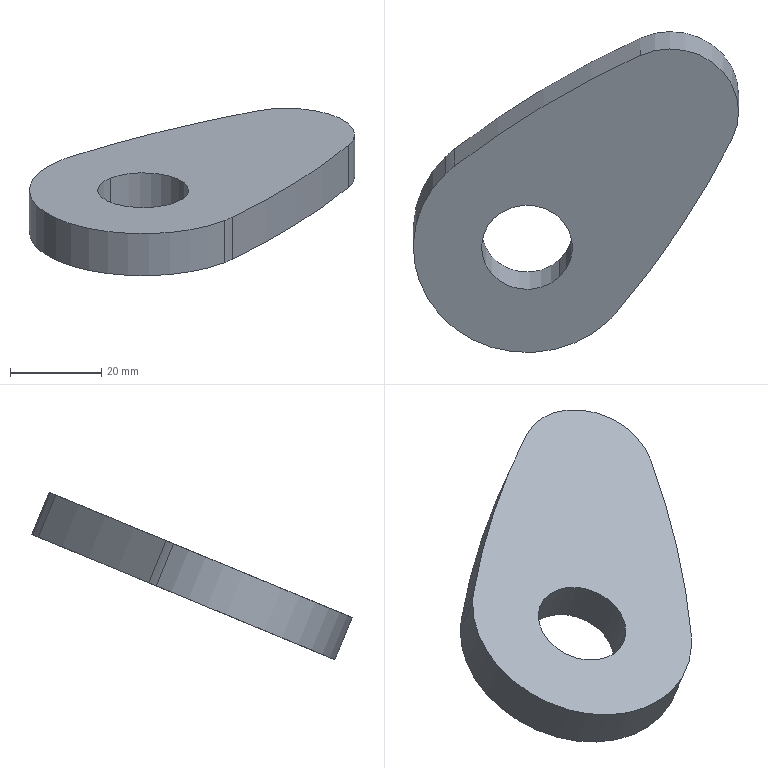Component | SolidWorks | Cam-1 | 1 solid | 10 faces | box 71.5 x 70.49 x 36.79 mm | volume 29441 mm3 | cylinder 8 | plane 2 | commonest cylinder face diameters 50 x3 20 x2 419.344 x2 30 x1
build123d program:
from build123d import *

# Parameters (mm, degrees)
BOSS_EXTRUDE1_DEPTH = 10
SKETCH2_R           = 10
CUT_EXTRUDE1_DEPTH  = 10


with BuildPart() as part:
    # Sketch1 → Boss-Extrude1 (new body)
    with BuildSketch(Plane.XY):
        with BuildLine():
            ThreePointArc((24.858, -2.66), (0, 25), (-24.858, -2.66))
            ThreePointArc((-24.858, -2.66), (-20.877, -26.632), (-14.149, -49.981))
            ThreePointArc((-14.149, -49.981), (0, -60), (14.149, -49.981))
            ThreePointArc((14.149, -49.981), (20.877, -26.632), (24.858, -2.66))
        make_face()
    extrude(amount=BOSS_EXTRUDE1_DEPTH)

    # Sketch2 → Cut-Extrude1 (cut)
    with BuildSketch(Plane.XY.offset(10)):
        Circle(SKETCH2_R)
    extrude(amount=-CUT_EXTRUDE1_DEPTH, mode=Mode.SUBTRACT)


solid = part.part

# Placed as in the assembly
solid = solid.moved(Location((-36.329, -1.596, 21.215), (-157.552, 0, 44.427)))
STEP:
#1=COLOUR_RGB('',0.7922,0.8196,0.9333);
#2=FILL_AREA_STYLE_COLOUR('',#1);
#3=FILL_AREA_STYLE('',(#2));
#4=SURFACE_STYLE_FILL_AREA(#3);
#5=SURFACE_SIDE_STYLE('',(#4));
#6=SURFACE_STYLE_USAGE(.BOTH.,#5);
#7=PRESENTATION_STYLE_ASSIGNMENT((#6));
#8=CARTESIAN_POINT('',(-1.149,-0.1672,0.3661));
#9=VERTEX_POINT('',#8);
#10=CARTESIAN_POINT('',(-1.711,0.3422,0.5766));
#11=VERTEX_POINT('',#10);
#12=CARTESIAN_POINT('',(-1.43,0.08749,0.4714));
#13=DIRECTION('',(-0.,-0.3818,0.9242));
#14=DIRECTION('',(-0.7141,0.647,0.2673));
#15=AXIS2_PLACEMENT_3D('',#12,#13,#14);
#16=CIRCLE('',#15,0.3937);
#17=EDGE_CURVE('',#9,#11,#16,.T.);
#18=ORIENTED_EDGE('',*,*,#17,.F.);
#19=CARTESIAN_POINT('',(-1.149,-0.3176,0.73));
#20=VERTEX_POINT('',#19);
#21=CARTESIAN_POINT('',(-1.149,-0.1672,0.3661));
#22=DIRECTION('',(-0.,-0.3818,0.9242));
#23=VECTOR('',#22,39.37);
#24=LINE('',#21,#23);
#25=EDGE_CURVE('',#9,#20,#24,.T.);
#26=ORIENTED_EDGE('',*,*,#25,.T.);
#27=CARTESIAN_POINT('',(-1.711,0.1919,0.9405));
#28=VERTEX_POINT('',#27);
#29=CARTESIAN_POINT('',(-1.43,-0.06285,0.8352));
#30=DIRECTION('',(-0.,-0.3818,0.9242));
#31=DIRECTION('',(-0.7141,0.647,0.2673));
#32=AXIS2_PLACEMENT_3D('',#29,#30,#31);
#33=CIRCLE('',#32,0.3937);
#34=EDGE_CURVE('',#20,#28,#33,.T.);
#35=ORIENTED_EDGE('',*,*,#34,.T.);
#36=CARTESIAN_POINT('',(-1.711,0.3422,0.5766));
#37=DIRECTION('',(-0.,-0.3818,0.9242));
#38=VECTOR('',#37,39.37);
#39=LINE('',#36,#38);
#40=EDGE_CURVE('',#11,#28,#39,.T.);
#41=ORIENTED_EDGE('',*,*,#40,.F.);
#42=EDGE_LOOP('',(#18,#26,#35,#41));
#43=FACE_OUTER_BOUND('',#42,.T.);
#44=CARTESIAN_POINT('',(-1.43,0.08749,0.4714));
#45=DIRECTION('',(-0.,-0.3818,0.9242));
#46=DIRECTION('',(-0.7141,0.647,0.2673));
#47=AXIS2_PLACEMENT_3D('',#44,#45,#46);
#48=CYLINDRICAL_SURFACE('',#47,0.3937);
#49=ADVANCED_FACE('',(#43),#48,.F.);
#50=CARTESIAN_POINT('',(-2.133,0.5739,1.098));
#51=VERTEX_POINT('',#50);
#52=CARTESIAN_POINT('',(-0.7274,-0.6996,0.5721));
#53=VERTEX_POINT('',#52);
#54=CARTESIAN_POINT('',(-1.43,-0.06285,0.8352));
#55=DIRECTION('',(-0.,-0.3818,0.9242));
#56=DIRECTION('',(-0.7141,0.647,0.2673));
#57=AXIS2_PLACEMENT_3D('',#54,#55,#56);
#58=CIRCLE('',#57,0.9843);
#59=EDGE_CURVE('',#51,#53,#58,.T.);
#60=ORIENTED_EDGE('',*,*,#59,.F.);
#61=CARTESIAN_POINT('',(-2.133,0.7243,0.7344));
#62=VERTEX_POINT('',#61);
#63=CARTESIAN_POINT('',(-2.133,0.5739,1.098));
#64=DIRECTION('',(0.,0.3818,-0.9242));
#65=VECTOR('',#64,39.37);
#66=LINE('',#63,#65);
#67=EDGE_CURVE('',#51,#62,#66,.T.);
#68=ORIENTED_EDGE('',*,*,#67,.T.);
#69=CARTESIAN_POINT('',(-0.7274,-0.5493,0.2083));
#70=VERTEX_POINT('',#69);
#71=CARTESIAN_POINT('',(-1.43,0.08749,0.4714));
#72=DIRECTION('',(-0.,-0.3818,0.9242));
#73=DIRECTION('',(-0.7141,0.647,0.2673));
#74=AXIS2_PLACEMENT_3D('',#71,#72,#73);
#75=CIRCLE('',#74,0.9843);
#76=EDGE_CURVE('',#62,#70,#75,.T.);
#77=ORIENTED_EDGE('',*,*,#76,.T.);
#78=CARTESIAN_POINT('',(-0.7274,-0.6996,0.5721));
#79=DIRECTION('',(0.,0.3818,-0.9242));
#80=VECTOR('',#79,39.37);
#81=LINE('',#78,#80);
#82=EDGE_CURVE('',#53,#70,#81,.T.);
#83=ORIENTED_EDGE('',*,*,#82,.F.);
#84=EDGE_LOOP('',(#60,#68,#77,#83));
#85=FACE_OUTER_BOUND('',#84,.T.);
#86=CARTESIAN_POINT('',(-1.43,-0.06285,0.8352));
#87=DIRECTION('',(0.,0.3818,-0.9242));
#88=DIRECTION('',(0.7141,-0.647,-0.2673));
#89=AXIS2_PLACEMENT_3D('',#86,#87,#88);
#90=CYLINDRICAL_SURFACE('',#89,0.9843);
#91=ADVANCED_FACE('',(#85),#90,.T.);
#92=CARTESIAN_POINT('',(-0.6581,-0.6269,0.6022));
#93=VERTEX_POINT('',#92);
#94=CARTESIAN_POINT('',(-1.43,-0.06285,0.8352));
#95=DIRECTION('',(-0.,-0.3818,0.9242));
#96=DIRECTION('',(-0.7141,0.647,0.2673));
#97=AXIS2_PLACEMENT_3D('',#94,#95,#96);
#98=CIRCLE('',#97,0.9843);
#99=EDGE_CURVE('',#53,#93,#98,.T.);
#100=ORIENTED_EDGE('',*,*,#99,.F.);
#101=ORIENTED_EDGE('',*,*,#82,.T.);
#102=CARTESIAN_POINT('',(-0.6581,-0.4765,0.2383));
#103=VERTEX_POINT('',#102);
#104=CARTESIAN_POINT('',(-1.43,0.08749,0.4714));
#105=DIRECTION('',(-0.,-0.3818,0.9242));
#106=DIRECTION('',(-0.7141,0.647,0.2673));
#107=AXIS2_PLACEMENT_3D('',#104,#105,#106);
#108=CIRCLE('',#107,0.9843);
#109=EDGE_CURVE('',#70,#103,#108,.T.);
#110=ORIENTED_EDGE('',*,*,#109,.T.);
#111=CARTESIAN_POINT('',(-0.6581,-0.6269,0.6022));
#112=DIRECTION('',(0.,0.3818,-0.9242));
#113=VECTOR('',#112,39.37);
#114=LINE('',#111,#113);
#115=EDGE_CURVE('',#93,#103,#114,.T.);
#116=ORIENTED_EDGE('',*,*,#115,.F.);
#117=EDGE_LOOP('',(#100,#101,#110,#116));
#118=FACE_OUTER_BOUND('',#117,.T.);
#119=CARTESIAN_POINT('',(-1.43,-0.06285,0.8352));
#120=DIRECTION('',(0.,0.3818,-0.9242));
#121=DIRECTION('',(0.7141,-0.647,-0.2673));
#122=AXIS2_PLACEMENT_3D('',#119,#120,#121);
#123=CYLINDRICAL_SURFACE('',#122,0.9843);
#124=ADVANCED_FACE('',(#118),#123,.T.);
#125=CARTESIAN_POINT('',(0.345,1.026,0.8591));
#126=VERTEX_POINT('',#125);
#127=CARTESIAN_POINT('',(-7.135,4.254,2.193));
#128=DIRECTION('',(-0.,-0.3818,0.9242));
#129=DIRECTION('',(-0.7141,0.647,0.2673));
#130=AXIS2_PLACEMENT_3D('',#127,#128,#129);
#131=CIRCLE('',#130,8.255);
#132=EDGE_CURVE('',#103,#126,#131,.T.);
#133=ORIENTED_EDGE('',*,*,#132,.T.);
#134=CARTESIAN_POINT('',(0.345,0.8756,1.223));
#135=VERTEX_POINT('',#134);
#136=CARTESIAN_POINT('',(0.345,0.8756,1.223));
#137=DIRECTION('',(0.,0.3818,-0.9242));
#138=VECTOR('',#137,39.37);
#139=LINE('',#136,#138);
#140=EDGE_CURVE('',#135,#126,#139,.T.);
#141=ORIENTED_EDGE('',*,*,#140,.F.);
#142=CARTESIAN_POINT('',(-7.135,4.104,2.557));
#143=DIRECTION('',(-0.,-0.3818,0.9242));
#144=DIRECTION('',(-0.7141,0.647,0.2673));
#145=AXIS2_PLACEMENT_3D('',#142,#143,#144);
#146=CIRCLE('',#145,8.255);
#147=EDGE_CURVE('',#93,#135,#146,.T.);
#148=ORIENTED_EDGE('',*,*,#147,.F.);
#149=ORIENTED_EDGE('',*,*,#115,.T.);
#150=EDGE_LOOP('',(#133,#141,#148,#149));
#151=FACE_OUTER_BOUND('',#150,.T.);
#152=CARTESIAN_POINT('',(-7.135,4.104,2.557));
#153=DIRECTION('',(0.,0.3818,-0.9242));
#154=DIRECTION('',(0.7141,-0.647,-0.2673));
#155=AXIS2_PLACEMENT_3D('',#152,#153,#154);
#156=CYLINDRICAL_SURFACE('',#155,8.255);
#157=ADVANCED_FACE('',(#151),#156,.T.);
#158=CARTESIAN_POINT('',(-0.4506,1.747,1.157));
#159=VERTEX_POINT('',#158);
#160=CARTESIAN_POINT('',(-0.1901,1.257,0.9545));
#161=DIRECTION('',(-0.,-0.3818,0.9242));
#162=DIRECTION('',(-0.7141,0.647,0.2673));
#163=AXIS2_PLACEMENT_3D('',#160,#161,#162);
#164=CIRCLE('',#163,0.5906);
#165=EDGE_CURVE('',#126,#159,#164,.T.);
#166=ORIENTED_EDGE('',*,*,#165,.T.);
#167=CARTESIAN_POINT('',(-0.4506,1.596,1.521));
#168=VERTEX_POINT('',#167);
#169=CARTESIAN_POINT('',(-0.4506,1.596,1.521));
#170=DIRECTION('',(0.,0.3818,-0.9242));
#171=VECTOR('',#170,39.37);
#172=LINE('',#169,#171);
#173=EDGE_CURVE('',#168,#159,#172,.T.);
#174=ORIENTED_EDGE('',*,*,#173,.F.);
#175=CARTESIAN_POINT('',(-0.1901,1.107,1.318));
#176=DIRECTION('',(-0.,-0.3818,0.9242));
#177=DIRECTION('',(-0.7141,0.647,0.2673));
#178=AXIS2_PLACEMENT_3D('',#175,#176,#177);
#179=CIRCLE('',#178,0.5906);
#180=EDGE_CURVE('',#135,#168,#179,.T.);
#181=ORIENTED_EDGE('',*,*,#180,.F.);
#182=ORIENTED_EDGE('',*,*,#140,.T.);
#183=EDGE_LOOP('',(#166,#174,#181,#182));
#184=FACE_OUTER_BOUND('',#183,.T.);
#185=CARTESIAN_POINT('',(-0.1901,1.107,1.318));
#186=DIRECTION('',(0.,0.3818,-0.9242));
#187=DIRECTION('',(0.7141,-0.647,-0.2673));
#188=AXIS2_PLACEMENT_3D('',#185,#186,#187);
#189=CYLINDRICAL_SURFACE('',#188,0.5906);
#190=ADVANCED_FACE('',(#184),#189,.T.);
#191=CARTESIAN_POINT('',(-2.056,0.7898,0.7615));
#192=VERTEX_POINT('',#191);
#193=CARTESIAN_POINT('',(3.191,-5.1,-1.672));
#194=DIRECTION('',(-0.,-0.3818,0.9242));
#195=DIRECTION('',(0.7141,-0.647,-0.2673));
#196=AXIS2_PLACEMENT_3D('',#193,#194,#195);
#197=CIRCLE('',#196,8.255);
#198=EDGE_CURVE('',#159,#192,#197,.T.);
#199=ORIENTED_EDGE('',*,*,#198,.T.);
#200=CARTESIAN_POINT('',(-2.056,0.6394,1.125));
#201=VERTEX_POINT('',#200);
#202=CARTESIAN_POINT('',(-2.056,0.6394,1.125));
#203=DIRECTION('',(0.,0.3818,-0.9242));
#204=VECTOR('',#203,39.37);
#205=LINE('',#202,#204);
#206=EDGE_CURVE('',#201,#192,#205,.T.);
#207=ORIENTED_EDGE('',*,*,#206,.F.);
#208=CARTESIAN_POINT('',(3.191,-5.25,-1.308));
#209=DIRECTION('',(-0.,-0.3818,0.9242));
#210=DIRECTION('',(0.7141,-0.647,-0.2673));
#211=AXIS2_PLACEMENT_3D('',#208,#209,#210);
#212=CIRCLE('',#211,8.255);
#213=EDGE_CURVE('',#168,#201,#212,.T.);
#214=ORIENTED_EDGE('',*,*,#213,.F.);
#215=ORIENTED_EDGE('',*,*,#173,.T.);
#216=EDGE_LOOP('',(#199,#207,#214,#215));
#217=FACE_OUTER_BOUND('',#216,.T.);
#218=CARTESIAN_POINT('',(3.191,-5.25,-1.308));
#219=DIRECTION('',(0.,0.3818,-0.9242));
#220=DIRECTION('',(0.7141,-0.647,-0.2673));
#221=AXIS2_PLACEMENT_3D('',#218,#219,#220);
#222=CYLINDRICAL_SURFACE('',#221,8.255);
#223=ADVANCED_FACE('',(#217),#222,.T.);
#224=ORIENTED_EDGE('',*,*,#67,.F.);
#225=CARTESIAN_POINT('',(-1.43,-0.06285,0.8352));
#226=DIRECTION('',(-0.,-0.3818,0.9242));
#227=DIRECTION('',(-0.7141,0.647,0.2673));
#228=AXIS2_PLACEMENT_3D('',#225,#226,#227);
#229=CIRCLE('',#228,0.9843);
#230=EDGE_CURVE('',#201,#51,#229,.T.);
#231=ORIENTED_EDGE('',*,*,#230,.F.);
#232=ORIENTED_EDGE('',*,*,#206,.T.);
#233=CARTESIAN_POINT('',(-1.43,0.08749,0.4714));
#234=DIRECTION('',(-0.,-0.3818,0.9242));
#235=DIRECTION('',(-0.7141,0.647,0.2673));
#236=AXIS2_PLACEMENT_3D('',#233,#234,#235);
#237=CIRCLE('',#236,0.9843);
#238=EDGE_CURVE('',#192,#62,#237,.T.);
#239=ORIENTED_EDGE('',*,*,#238,.T.);
#240=EDGE_LOOP('',(#224,#231,#232,#239));
#241=FACE_OUTER_BOUND('',#240,.T.);
#242=CARTESIAN_POINT('',(-1.43,-0.06285,0.8352));
#243=DIRECTION('',(0.,0.3818,-0.9242));
#244=DIRECTION('',(0.7141,-0.647,-0.2673));
#245=AXIS2_PLACEMENT_3D('',#242,#243,#244);
#246=CYLINDRICAL_SURFACE('',#245,0.9843);
#247=ADVANCED_FACE('',(#241),#246,.T.);
#248=CARTESIAN_POINT('',(-1.43,-0.06285,0.8352));
#249=DIRECTION('',(-0.,-0.3818,0.9242));
#250=DIRECTION('',(-0.7141,0.647,0.2673));
#251=AXIS2_PLACEMENT_3D('',#248,#249,#250);
#252=CIRCLE('',#251,0.3937);
#253=EDGE_CURVE('',#28,#20,#252,.T.);
#254=ORIENTED_EDGE('',*,*,#253,.F.);
#255=ORIENTED_EDGE('',*,*,#34,.F.);
#256=EDGE_LOOP('',(#254,#255));
#257=FACE_BOUND('',#256,.T.);
#258=ORIENTED_EDGE('',*,*,#147,.T.);
#259=ORIENTED_EDGE('',*,*,#180,.T.);
#260=ORIENTED_EDGE('',*,*,#213,.T.);
#261=ORIENTED_EDGE('',*,*,#230,.T.);
#262=ORIENTED_EDGE('',*,*,#59,.T.);
#263=ORIENTED_EDGE('',*,*,#99,.T.);
#264=EDGE_LOOP('',(#258,#259,#260,#261,#262,#263));
#265=FACE_OUTER_BOUND('',#264,.T.);
#266=CARTESIAN_POINT('',(-3.662,2.605,1.937));
#267=DIRECTION('',(-0.,-0.3818,0.9242));
#268=DIRECTION('',(-0.7141,0.647,0.2673));
#269=AXIS2_PLACEMENT_3D('',#266,#267,#268);
#270=PLANE('',#269);
#271=ADVANCED_FACE('',(#257,#265),#270,.T.);
#272=CARTESIAN_POINT('',(-1.43,0.08749,0.4714));
#273=DIRECTION('',(-0.,-0.3818,0.9242));
#274=DIRECTION('',(-0.7141,0.647,0.2673));
#275=AXIS2_PLACEMENT_3D('',#272,#273,#274);
#276=CIRCLE('',#275,0.3937);
#277=EDGE_CURVE('',#11,#9,#276,.T.);
#278=ORIENTED_EDGE('',*,*,#277,.T.);
#279=ORIENTED_EDGE('',*,*,#17,.T.);
#280=EDGE_LOOP('',(#278,#279));
#281=FACE_BOUND('',#280,.T.);
#282=ORIENTED_EDGE('',*,*,#132,.F.);
#283=ORIENTED_EDGE('',*,*,#109,.F.);
#284=ORIENTED_EDGE('',*,*,#76,.F.);
#285=ORIENTED_EDGE('',*,*,#238,.F.);
#286=ORIENTED_EDGE('',*,*,#198,.F.);
#287=ORIENTED_EDGE('',*,*,#165,.F.);
#288=EDGE_LOOP('',(#282,#283,#284,#285,#286,#287));
#289=FACE_OUTER_BOUND('',#288,.T.);
#290=CARTESIAN_POINT('',(-3.662,2.755,1.574));
#291=DIRECTION('',(-0.,-0.3818,0.9242));
#292=DIRECTION('',(-0.7141,0.647,0.2673));
#293=AXIS2_PLACEMENT_3D('',#290,#291,#292);
#294=PLANE('',#293);
#295=ADVANCED_FACE('',(#281,#289),#294,.F.);
#296=ORIENTED_EDGE('',*,*,#25,.F.);
#297=ORIENTED_EDGE('',*,*,#277,.F.);
#298=ORIENTED_EDGE('',*,*,#40,.T.);
#299=ORIENTED_EDGE('',*,*,#253,.T.);
#300=EDGE_LOOP('',(#296,#297,#298,#299));
#301=FACE_OUTER_BOUND('',#300,.T.);
#302=CARTESIAN_POINT('',(-1.43,0.08749,0.4714));
#303=DIRECTION('',(-0.,-0.3818,0.9242));
#304=DIRECTION('',(-0.7141,0.647,0.2673));
#305=AXIS2_PLACEMENT_3D('',#302,#303,#304);
#306=CYLINDRICAL_SURFACE('',#305,0.3937);
#307=ADVANCED_FACE('',(#301),#306,.F.);
#308=CLOSED_SHELL('',(#49,#91,#124,#157,#190,#223,#247,#271,#295,#307));
#309=MANIFOLD_SOLID_BREP('',#308);
#310=STYLED_ITEM('',(#7),#309);
#311=PRESENTATION_LAYER_ASSIGNMENT('','',(#310));
#312=(LENGTH_UNIT()NAMED_UNIT(*)SI_UNIT($,.METRE.));
#313=LENGTH_MEASURE_WITH_UNIT(LENGTH_MEASURE(0.0254),#312);
#314=DIMENSIONAL_EXPONENTS(1.,0.,0.,0.,0.,0.,0.);
#315=(CONVERSION_BASED_UNIT('',#313)LENGTH_UNIT()NAMED_UNIT(#314));
#316=UNCERTAINTY_MEASURE_WITH_UNIT(LENGTH_MEASURE(0.00001),#315,'','');
#317=(NAMED_UNIT(*)PLANE_ANGLE_UNIT()SI_UNIT($,.RADIAN.));
#318=(NAMED_UNIT(*)SI_UNIT($,.STERADIAN.)SOLID_ANGLE_UNIT());
#319=(GEOMETRIC_REPRESENTATION_CONTEXT(3)GLOBAL_UNCERTAINTY_ASSIGNED_CONTEXT((#316))GLOBAL_UNIT_ASSIGNED_CONTEXT((#315,#317,#318))REPRESENTATION_CONTEXT('',''));
#320=MECHANICAL_DESIGN_GEOMETRIC_PRESENTATION_REPRESENTATION('',(#310),#319);
#321=CARTESIAN_POINT('',(0.,0.,0.));
#322=DIRECTION('',(0.,0.,1.));
#323=DIRECTION('',(1.,0.,0.));
#324=AXIS2_PLACEMENT_3D('',#321,#322,#323);
#325=(LENGTH_UNIT()NAMED_UNIT(*)SI_UNIT($,.METRE.));
#326=LENGTH_MEASURE_WITH_UNIT(LENGTH_MEASURE(0.0254),#325);
#327=DIMENSIONAL_EXPONENTS(1.,0.,0.,0.,0.,0.,0.);
#328=(CONVERSION_BASED_UNIT('',#326)LENGTH_UNIT()NAMED_UNIT(#327));
#329=UNCERTAINTY_MEASURE_WITH_UNIT(LENGTH_MEASURE(0.00001),#328,'','');
#330=(NAMED_UNIT(*)PLANE_ANGLE_UNIT()SI_UNIT($,.RADIAN.));
#331=(NAMED_UNIT(*)SI_UNIT($,.STERADIAN.)SOLID_ANGLE_UNIT());
#332=(GEOMETRIC_REPRESENTATION_CONTEXT(3)GLOBAL_UNCERTAINTY_ASSIGNED_CONTEXT((#329))GLOBAL_UNIT_ASSIGNED_CONTEXT((#328,#330,#331))REPRESENTATION_CONTEXT('',''));
#333=ADVANCED_BREP_SHAPE_REPRESENTATION('',(#309,#324),#332);